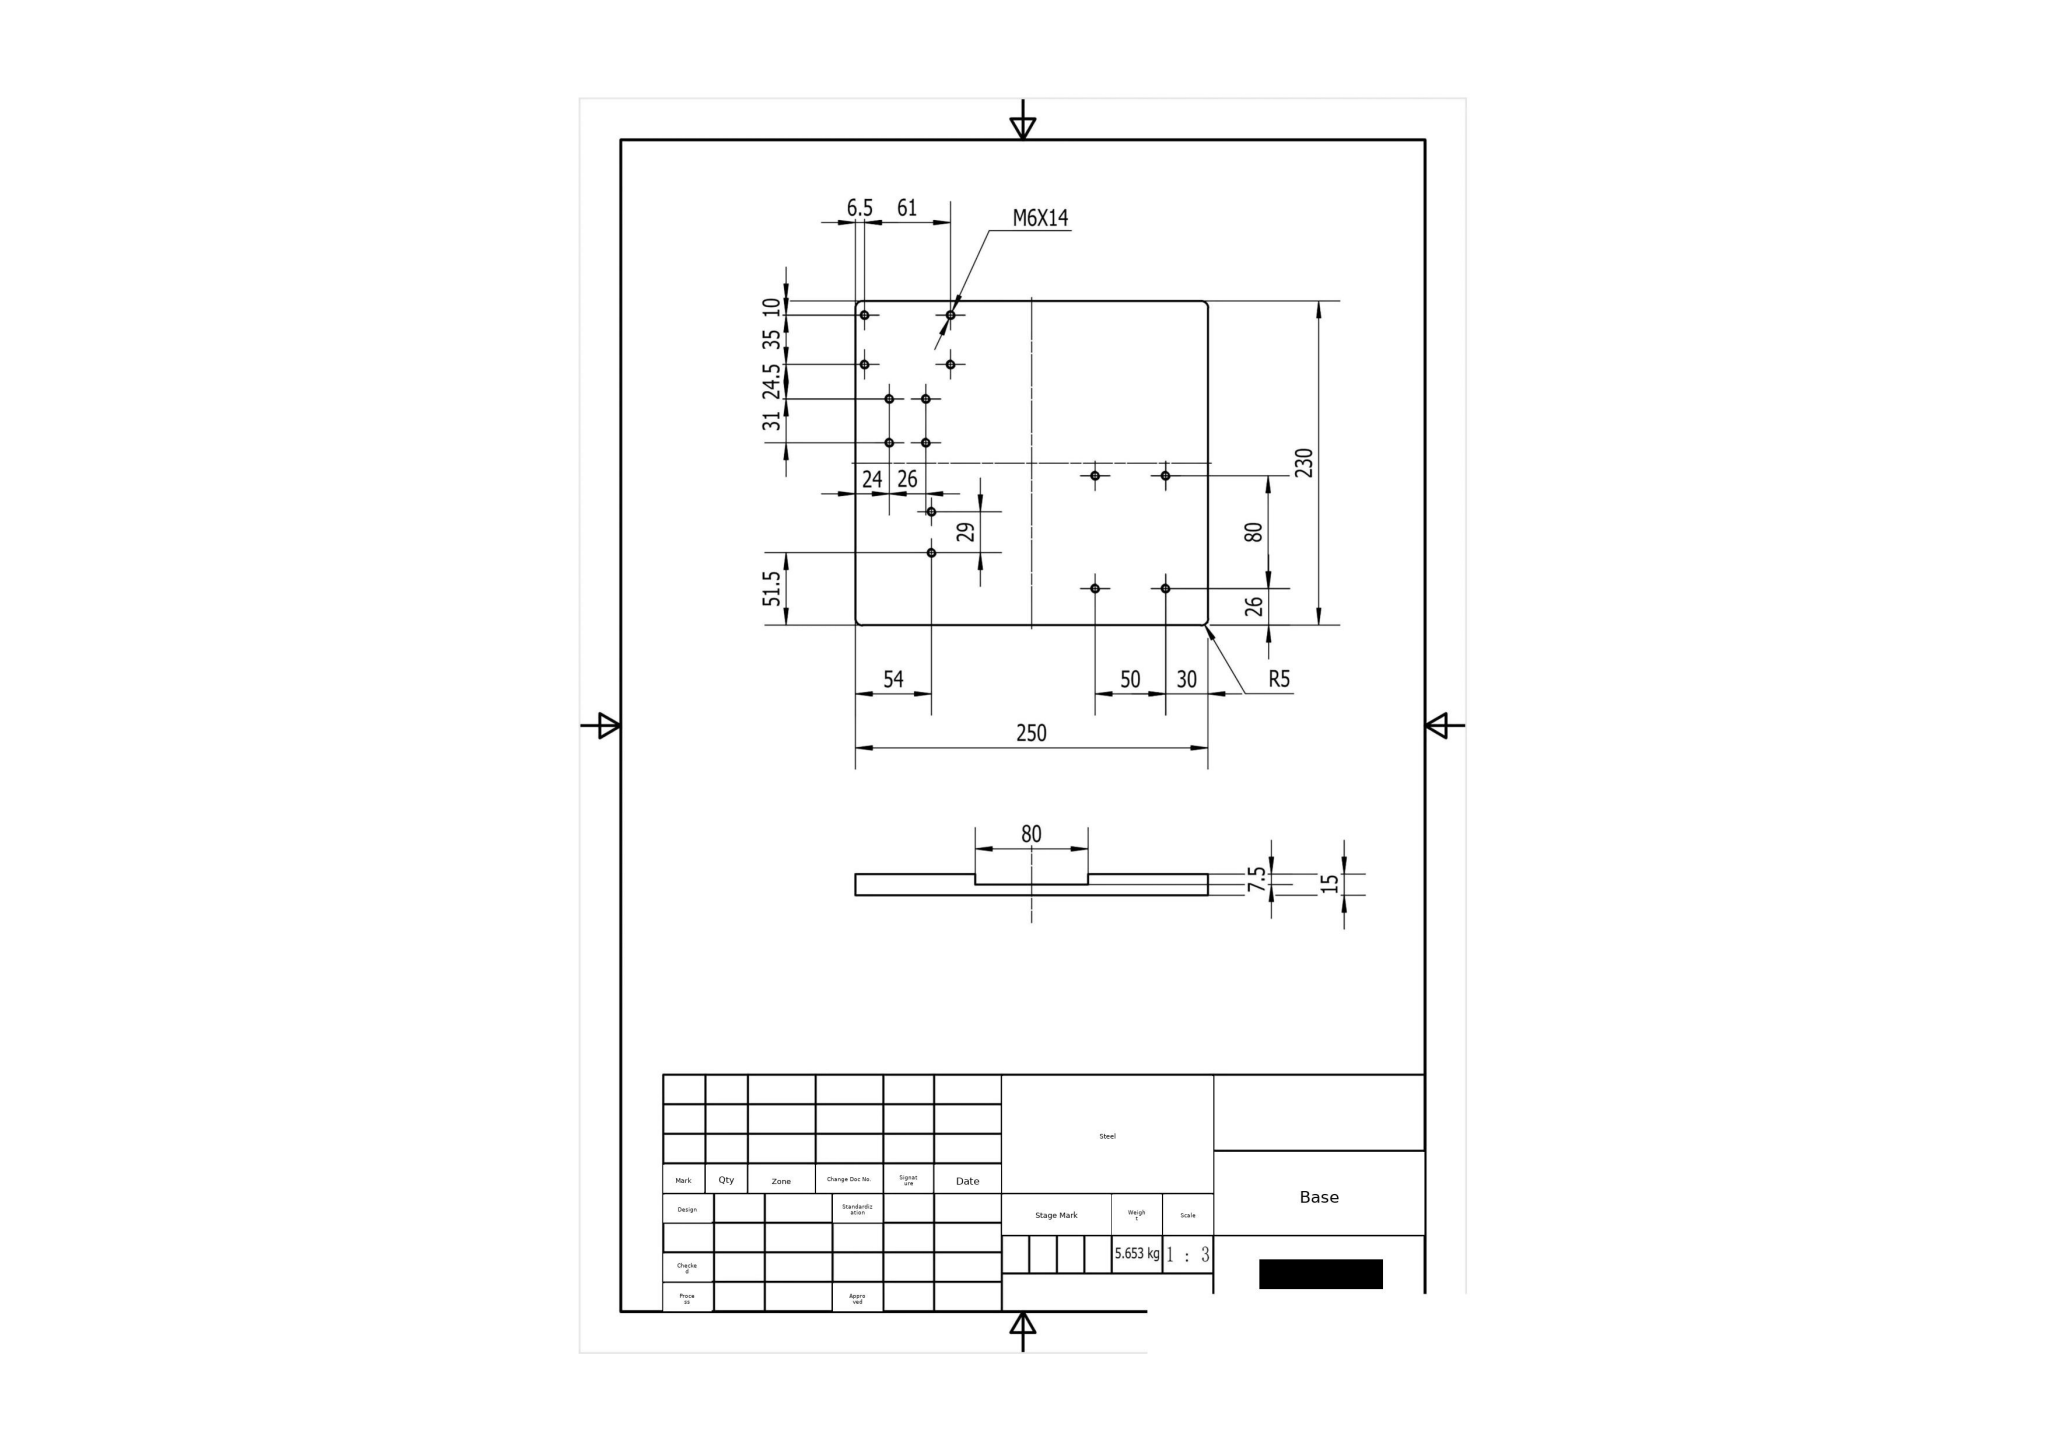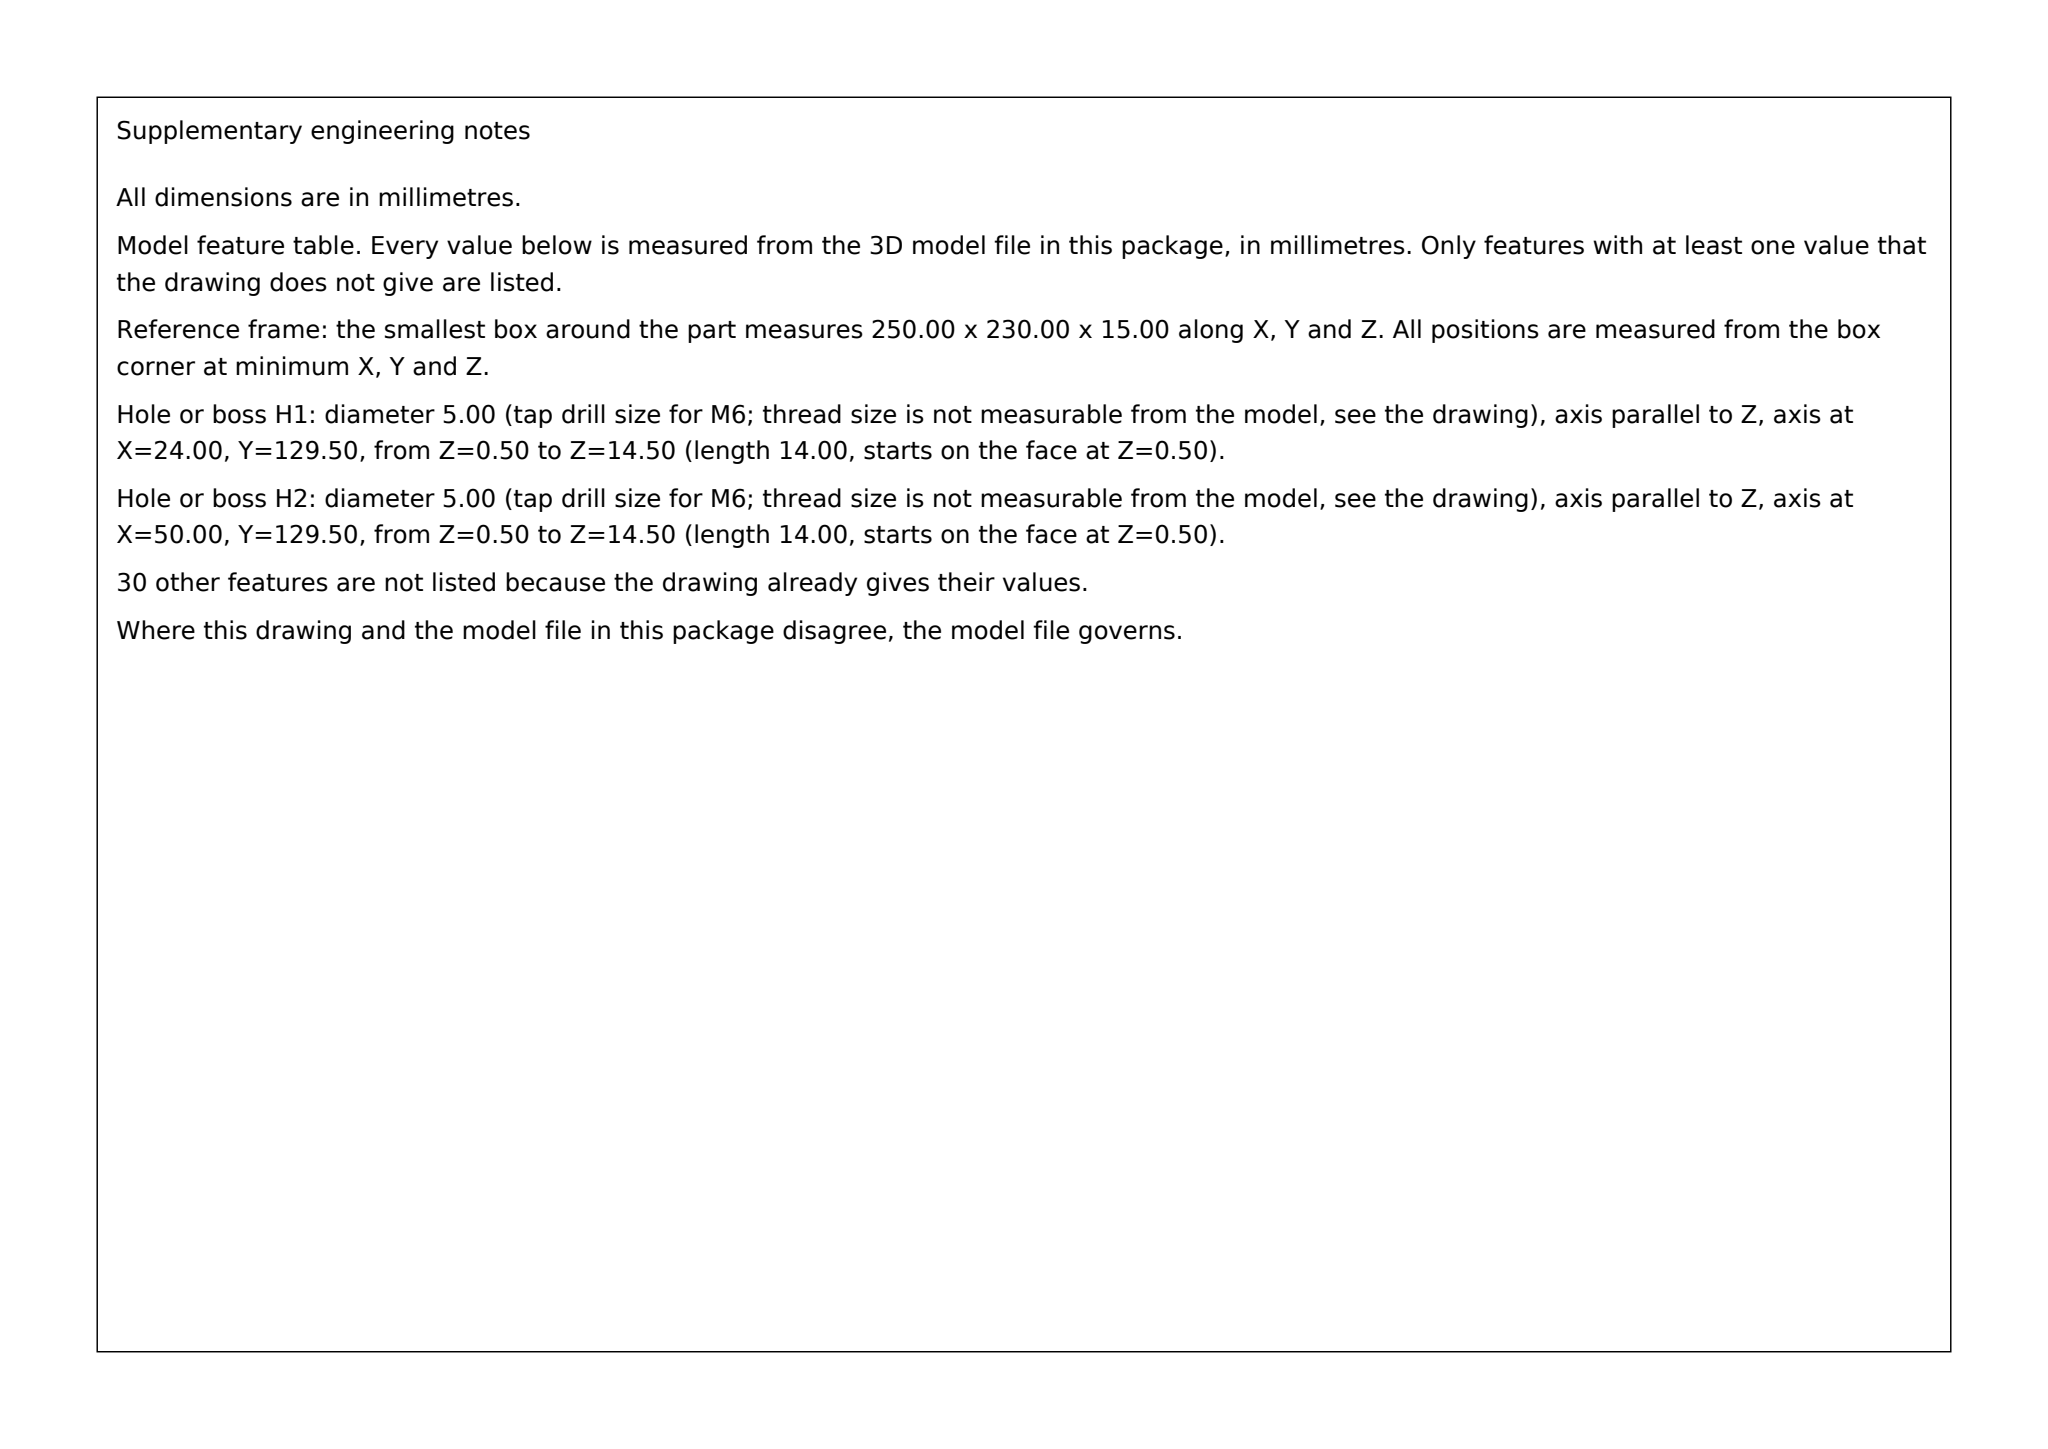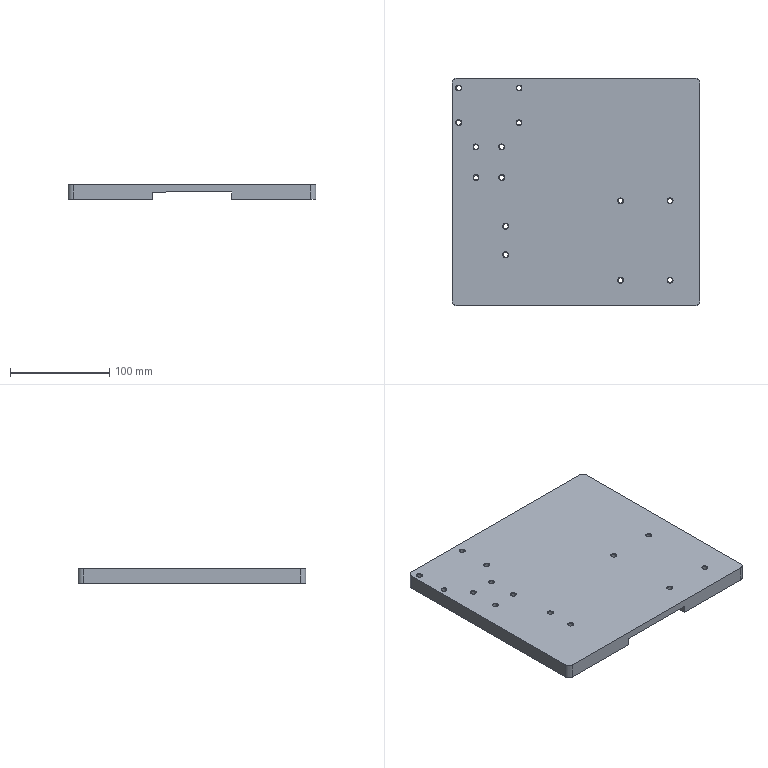Part | SolidWorks | mm | material Steel | 1 solid | 98 faces | box 250 x 230 x 15 mm | volume 719996 mm3 | cone 56 | cylinder 32 | plane 10 | commonest cylinder face diameters 5 x28 10 x4